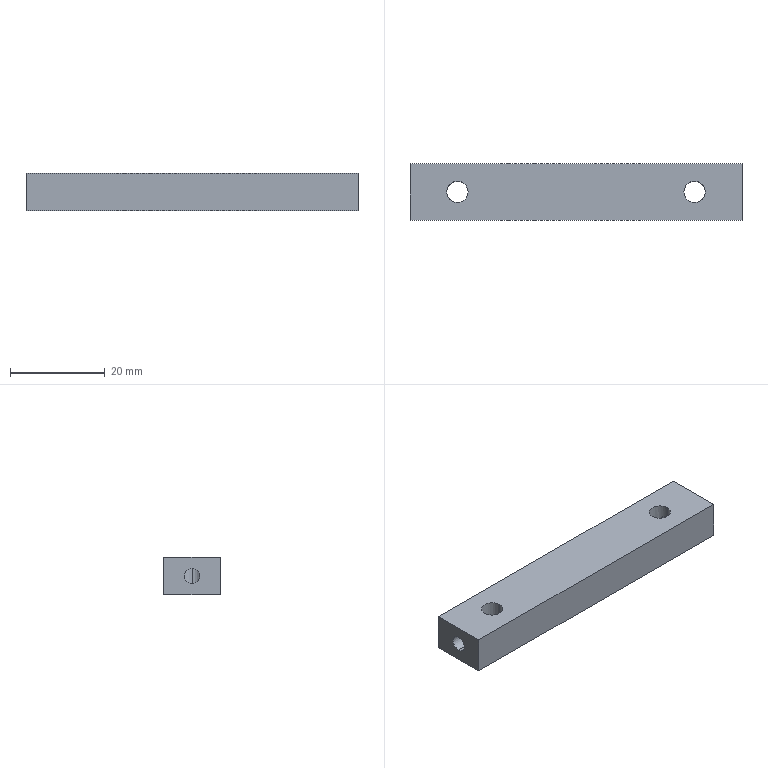Component | SolidWorks | InnerBagLiftingAluminumBlockB-1 | 1 solid | 14 faces | box 70 x 12 x 8 mm | volume 6330 mm3 | cylinder 8 | plane 6 | commonest cylinder face diameters 3.3 x4 4.5 x4
build123d program:
from build123d import *

# Parameters (mm, degrees)
SKETCH1_W             = 70
SKETCH1_H             = 12
BOSS_EXTRUDE1_DEPTH   = 4
SKETCH2_R             = 2.25
CUT_EXTRUDE1_DEPTH    = 8
M4_TAPPED_HOLE1_D     = 3.3
M4_TAPPED_HOLE1_DEPTH = 10.1
M4_TAPPED_HOLE1_TIP   = 1.65
M4_TAPPED_HOLE2_D     = 3.3
M4_TAPPED_HOLE2_DEPTH = 10.1
M4_TAPPED_HOLE2_TIP   = 1.65


with BuildPart() as part:
    # Sketch1 → Boss-Extrude1 (new, symmetric)
    with BuildSketch(Plane.XY):
        with Locations((35, 6)):
            Rectangle(SKETCH1_W, SKETCH1_H)
    extrude(amount=BOSS_EXTRUDE1_DEPTH, both=True)

    # Sketch2 → Cut-Extrude1 (cut)
    with BuildSketch(Plane.XY.offset(4)):
        with Locations((10, 6)):
            Circle(SKETCH2_R)
        with Locations((60, 6)):
            Circle(SKETCH2_R)
    extrude(amount=-CUT_EXTRUDE1_DEPTH, mode=Mode.SUBTRACT)

    # M4 Tapped Hole1
    with Locations(Plane(origin=(70, 6, 0), x_dir=(0, 0, 1), z_dir=(1, 0, 0))):
        with Locations((0, 0)):
            Hole(M4_TAPPED_HOLE1_D / 2, depth=M4_TAPPED_HOLE1_DEPTH)
            with Locations((0, 0, -(M4_TAPPED_HOLE1_DEPTH + M4_TAPPED_HOLE1_TIP / 2))):  # 90° drill point
                Cone(0, M4_TAPPED_HOLE1_D / 2, M4_TAPPED_HOLE1_TIP, mode=Mode.SUBTRACT)

    # M4 Tapped Hole2
    with Locations(Plane(origin=(0, 6, 0), x_dir=(0, 0, -1), z_dir=(-1, 0, 0))):
        with Locations((0, 0)):
            Hole(M4_TAPPED_HOLE2_D / 2, depth=M4_TAPPED_HOLE2_DEPTH)
            with Locations((0, 0, -(M4_TAPPED_HOLE2_DEPTH + M4_TAPPED_HOLE2_TIP / 2))):  # 90° drill point
                Cone(0, M4_TAPPED_HOLE2_D / 2, M4_TAPPED_HOLE2_TIP, mode=Mode.SUBTRACT)


solid = part.part

# Placed as in the assembly
solid = solid.moved(Location((29.354, -54.068, 191.933), (0, 0, 0)))
STEP:
#1=CARTESIAN_POINT('',(1.461,-1.892,7.491));
#2=VERTEX_POINT('',#1);
#3=CARTESIAN_POINT('',(1.461,-1.892,7.621));
#4=VERTEX_POINT('',#3);
#5=CARTESIAN_POINT('',(1.461,-1.892,7.491));
#6=CARTESIAN_POINT('',(1.461,-1.897,7.491));
#7=CARTESIAN_POINT('',(1.461,-1.901,7.492));
#8=CARTESIAN_POINT('',(1.462,-1.91,7.494));
#9=CARTESIAN_POINT('',(1.463,-1.914,7.495));
#10=CARTESIAN_POINT('',(1.467,-1.926,7.5));
#11=CARTESIAN_POINT('',(1.47,-1.933,7.505));
#12=CARTESIAN_POINT('',(1.477,-1.944,7.517));
#13=CARTESIAN_POINT('',(1.481,-1.949,7.523));
#14=CARTESIAN_POINT('',(1.487,-1.955,7.539));
#15=CARTESIAN_POINT('',(1.489,-1.957,7.547));
#16=CARTESIAN_POINT('',(1.489,-1.957,7.565));
#17=CARTESIAN_POINT('',(1.487,-1.955,7.574));
#18=CARTESIAN_POINT('',(1.483,-1.951,7.586));
#19=CARTESIAN_POINT('',(1.481,-1.949,7.589));
#20=CARTESIAN_POINT('',(1.477,-1.944,7.596));
#21=CARTESIAN_POINT('',(1.476,-1.941,7.599));
#22=CARTESIAN_POINT('',(1.472,-1.936,7.605));
#23=CARTESIAN_POINT('',(1.47,-1.933,7.608));
#24=CARTESIAN_POINT('',(1.467,-1.926,7.612));
#25=CARTESIAN_POINT('',(1.466,-1.922,7.614));
#26=CARTESIAN_POINT('',(1.462,-1.91,7.619));
#27=CARTESIAN_POINT('',(1.461,-1.901,7.621));
#28=CARTESIAN_POINT('',(1.461,-1.892,7.621));
#29=B_SPLINE_CURVE_WITH_KNOTS('',3,(#5,#6,#7,#8,#9,#10,#11,#12,#13,#14,#15,#16,#17,#18,#19,#20,#21,#22,#23,#24,#25,#26,#27,#28),.UNSPECIFIED.,.F.,.F.,(4,2,2,2,2,2,2,2,2,2,2,4),(0.005391,0.005727,0.006063,0.006736,0.007408,0.008081,0.008754,0.00909,0.009426,0.009762,0.0101,0.01077),.UNSPECIFIED.);
#30=EDGE_CURVE('',#2,#4,#29,.T.);
#31=ORIENTED_EDGE('',*,*,#30,.F.);
#32=CARTESIAN_POINT('',(1.156,-1.892,7.491));
#33=VERTEX_POINT('',#32);
#34=CARTESIAN_POINT('',(1.156,-1.892,7.491));
#35=DIRECTION('',(-1.,0.,0.));
#36=VECTOR('',#35,39.37);
#37=LINE('',#34,#36);
#38=EDGE_CURVE('',#2,#33,#37,.T.);
#39=ORIENTED_EDGE('',*,*,#38,.T.);
#40=CARTESIAN_POINT('',(1.156,-1.892,7.621));
#41=VERTEX_POINT('',#40);
#42=CARTESIAN_POINT('',(1.156,-1.892,7.556));
#43=DIRECTION('',(-1.,0.,0.));
#44=DIRECTION('',(0.,0.,1.));
#45=AXIS2_PLACEMENT_3D('',#42,#43,#44);
#46=CIRCLE('',#45,0.06496);
#47=EDGE_CURVE('',#33,#41,#46,.T.);
#48=ORIENTED_EDGE('',*,*,#47,.T.);
#49=CARTESIAN_POINT('',(1.156,-1.892,7.621));
#50=DIRECTION('',(-1.,0.,0.));
#51=VECTOR('',#50,39.37);
#52=LINE('',#49,#51);
#53=EDGE_CURVE('',#4,#41,#52,.T.);
#54=ORIENTED_EDGE('',*,*,#53,.F.);
#55=EDGE_LOOP('',(#31,#39,#48,#54));
#56=FACE_OUTER_BOUND('',#55,.T.);
#57=CARTESIAN_POINT('',(1.156,-1.892,7.556));
#58=DIRECTION('',(-1.,0.,0.));
#59=DIRECTION('',(0.,0.,1.));
#60=AXIS2_PLACEMENT_3D('',#57,#58,#59);
#61=CYLINDRICAL_SURFACE('',#60,0.06496);
#62=ADVANCED_FACE('',(#56),#61,.F.);
#63=CARTESIAN_POINT('',(3.606,-1.892,7.621));
#64=VERTEX_POINT('',#63);
#65=CARTESIAN_POINT('',(3.606,-1.892,7.491));
#66=VERTEX_POINT('',#65);
#67=CARTESIAN_POINT('',(3.606,-1.892,7.621));
#68=CARTESIAN_POINT('',(3.606,-1.897,7.621));
#69=CARTESIAN_POINT('',(3.606,-1.901,7.621));
#70=CARTESIAN_POINT('',(3.605,-1.91,7.619));
#71=CARTESIAN_POINT('',(3.604,-1.914,7.618));
#72=CARTESIAN_POINT('',(3.6,-1.926,7.613));
#73=CARTESIAN_POINT('',(3.597,-1.933,7.608));
#74=CARTESIAN_POINT('',(3.59,-1.944,7.596));
#75=CARTESIAN_POINT('',(3.586,-1.949,7.589));
#76=CARTESIAN_POINT('',(3.58,-1.955,7.574));
#77=CARTESIAN_POINT('',(3.578,-1.957,7.565));
#78=CARTESIAN_POINT('',(3.578,-1.957,7.547));
#79=CARTESIAN_POINT('',(3.58,-1.955,7.539));
#80=CARTESIAN_POINT('',(3.585,-1.951,7.527));
#81=CARTESIAN_POINT('',(3.586,-1.949,7.524));
#82=CARTESIAN_POINT('',(3.59,-1.944,7.517));
#83=CARTESIAN_POINT('',(3.592,-1.941,7.514));
#84=CARTESIAN_POINT('',(3.595,-1.936,7.508));
#85=CARTESIAN_POINT('',(3.597,-1.933,7.505));
#86=CARTESIAN_POINT('',(3.6,-1.926,7.5));
#87=CARTESIAN_POINT('',(3.601,-1.922,7.498));
#88=CARTESIAN_POINT('',(3.605,-1.91,7.493));
#89=CARTESIAN_POINT('',(3.606,-1.901,7.491));
#90=CARTESIAN_POINT('',(3.606,-1.892,7.491));
#91=B_SPLINE_CURVE_WITH_KNOTS('',3,(#67,#68,#69,#70,#71,#72,#73,#74,#75,#76,#77,#78,#79,#80,#81,#82,#83,#84,#85,#86,#87,#88,#89,#90),.UNSPECIFIED.,.F.,.F.,(4,2,2,2,2,2,2,2,2,2,2,4),(0.005391,0.005727,0.006063,0.006736,0.007408,0.008081,0.008754,0.00909,0.009426,0.009762,0.0101,0.01077),.UNSPECIFIED.);
#92=EDGE_CURVE('',#64,#66,#91,.T.);
#93=ORIENTED_EDGE('',*,*,#92,.F.);
#94=CARTESIAN_POINT('',(3.912,-1.892,7.621));
#95=VERTEX_POINT('',#94);
#96=CARTESIAN_POINT('',(3.912,-1.892,7.621));
#97=DIRECTION('',(1.,0.,0.));
#98=VECTOR('',#97,39.37);
#99=LINE('',#96,#98);
#100=EDGE_CURVE('',#64,#95,#99,.T.);
#101=ORIENTED_EDGE('',*,*,#100,.T.);
#102=CARTESIAN_POINT('',(3.912,-1.892,7.491));
#103=VERTEX_POINT('',#102);
#104=CARTESIAN_POINT('',(3.912,-1.892,7.556));
#105=DIRECTION('',(1.,0.,0.));
#106=DIRECTION('',(0.,0.,-1.));
#107=AXIS2_PLACEMENT_3D('',#104,#105,#106);
#108=CIRCLE('',#107,0.06496);
#109=EDGE_CURVE('',#95,#103,#108,.T.);
#110=ORIENTED_EDGE('',*,*,#109,.T.);
#111=CARTESIAN_POINT('',(3.912,-1.892,7.491));
#112=DIRECTION('',(1.,0.,0.));
#113=VECTOR('',#112,39.37);
#114=LINE('',#111,#113);
#115=EDGE_CURVE('',#66,#103,#114,.T.);
#116=ORIENTED_EDGE('',*,*,#115,.F.);
#117=EDGE_LOOP('',(#93,#101,#110,#116));
#118=FACE_OUTER_BOUND('',#117,.T.);
#119=CARTESIAN_POINT('',(3.912,-1.892,7.556));
#120=DIRECTION('',(1.,0.,0.));
#121=DIRECTION('',(0.,0.,-1.));
#122=AXIS2_PLACEMENT_3D('',#119,#120,#121);
#123=CYLINDRICAL_SURFACE('',#122,0.06496);
#124=ADVANCED_FACE('',(#118),#123,.F.);
#125=CARTESIAN_POINT('',(3.429,-1.892,7.399));
#126=VERTEX_POINT('',#125);
#127=CARTESIAN_POINT('',(3.606,-1.892,7.399));
#128=VERTEX_POINT('',#127);
#129=CARTESIAN_POINT('',(3.518,-1.892,7.399));
#130=DIRECTION('',(0.,0.,1.));
#131=DIRECTION('',(1.,0.,0.));
#132=AXIS2_PLACEMENT_3D('',#129,#130,#131);
#133=CIRCLE('',#132,0.08858);
#134=EDGE_CURVE('',#126,#128,#133,.T.);
#135=ORIENTED_EDGE('',*,*,#134,.F.);
#136=CARTESIAN_POINT('',(3.429,-1.892,7.714));
#137=VERTEX_POINT('',#136);
#138=CARTESIAN_POINT('',(3.429,-1.892,7.399));
#139=DIRECTION('',(0.,0.,1.));
#140=VECTOR('',#139,39.37);
#141=LINE('',#138,#140);
#142=EDGE_CURVE('',#126,#137,#141,.T.);
#143=ORIENTED_EDGE('',*,*,#142,.T.);
#144=CARTESIAN_POINT('',(3.606,-1.892,7.714));
#145=VERTEX_POINT('',#144);
#146=CARTESIAN_POINT('',(3.518,-1.892,7.714));
#147=DIRECTION('',(0.,0.,1.));
#148=DIRECTION('',(1.,0.,0.));
#149=AXIS2_PLACEMENT_3D('',#146,#147,#148);
#150=CIRCLE('',#149,0.08858);
#151=EDGE_CURVE('',#137,#145,#150,.T.);
#152=ORIENTED_EDGE('',*,*,#151,.T.);
#153=CARTESIAN_POINT('',(3.606,-1.892,7.399));
#154=DIRECTION('',(0.,0.,1.));
#155=VECTOR('',#154,39.37);
#156=LINE('',#153,#155);
#157=EDGE_CURVE('',#64,#145,#156,.T.);
#158=ORIENTED_EDGE('',*,*,#157,.F.);
#159=ORIENTED_EDGE('',*,*,#92,.T.);
#160=CARTESIAN_POINT('',(3.606,-1.892,7.399));
#161=DIRECTION('',(0.,0.,1.));
#162=VECTOR('',#161,39.37);
#163=LINE('',#160,#162);
#164=EDGE_CURVE('',#128,#66,#163,.T.);
#165=ORIENTED_EDGE('',*,*,#164,.F.);
#166=EDGE_LOOP('',(#135,#143,#152,#158,#159,#165));
#167=FACE_OUTER_BOUND('',#166,.T.);
#168=CARTESIAN_POINT('',(3.518,-1.892,7.399));
#169=DIRECTION('',(0.,0.,1.));
#170=DIRECTION('',(1.,0.,0.));
#171=AXIS2_PLACEMENT_3D('',#168,#169,#170);
#172=CYLINDRICAL_SURFACE('',#171,0.08858);
#173=ADVANCED_FACE('',(#167),#172,.F.);
#174=CARTESIAN_POINT('',(1.461,-1.892,7.399));
#175=VERTEX_POINT('',#174);
#176=CARTESIAN_POINT('',(1.638,-1.892,7.399));
#177=VERTEX_POINT('',#176);
#178=CARTESIAN_POINT('',(1.549,-1.892,7.399));
#179=DIRECTION('',(0.,0.,1.));
#180=DIRECTION('',(1.,0.,0.));
#181=AXIS2_PLACEMENT_3D('',#178,#179,#180);
#182=CIRCLE('',#181,0.08858);
#183=EDGE_CURVE('',#175,#177,#182,.T.);
#184=ORIENTED_EDGE('',*,*,#183,.F.);
#185=CARTESIAN_POINT('',(1.461,-1.892,7.399));
#186=DIRECTION('',(0.,0.,1.));
#187=VECTOR('',#186,39.37);
#188=LINE('',#185,#187);
#189=EDGE_CURVE('',#175,#2,#188,.T.);
#190=ORIENTED_EDGE('',*,*,#189,.T.);
#191=ORIENTED_EDGE('',*,*,#30,.T.);
#192=CARTESIAN_POINT('',(1.461,-1.892,7.714));
#193=VERTEX_POINT('',#192);
#194=CARTESIAN_POINT('',(1.461,-1.892,7.399));
#195=DIRECTION('',(0.,0.,1.));
#196=VECTOR('',#195,39.37);
#197=LINE('',#194,#196);
#198=EDGE_CURVE('',#4,#193,#197,.T.);
#199=ORIENTED_EDGE('',*,*,#198,.T.);
#200=CARTESIAN_POINT('',(1.638,-1.892,7.714));
#201=VERTEX_POINT('',#200);
#202=CARTESIAN_POINT('',(1.549,-1.892,7.714));
#203=DIRECTION('',(0.,0.,1.));
#204=DIRECTION('',(1.,0.,0.));
#205=AXIS2_PLACEMENT_3D('',#202,#203,#204);
#206=CIRCLE('',#205,0.08858);
#207=EDGE_CURVE('',#193,#201,#206,.T.);
#208=ORIENTED_EDGE('',*,*,#207,.T.);
#209=CARTESIAN_POINT('',(1.638,-1.892,7.399));
#210=DIRECTION('',(0.,0.,1.));
#211=VECTOR('',#210,39.37);
#212=LINE('',#209,#211);
#213=EDGE_CURVE('',#177,#201,#212,.T.);
#214=ORIENTED_EDGE('',*,*,#213,.F.);
#215=EDGE_LOOP('',(#184,#190,#191,#199,#208,#214));
#216=FACE_OUTER_BOUND('',#215,.T.);
#217=CARTESIAN_POINT('',(1.549,-1.892,7.399));
#218=DIRECTION('',(0.,0.,1.));
#219=DIRECTION('',(1.,0.,0.));
#220=AXIS2_PLACEMENT_3D('',#217,#218,#219);
#221=CYLINDRICAL_SURFACE('',#220,0.08858);
#222=ADVANCED_FACE('',(#216),#221,.F.);
#223=CARTESIAN_POINT('',(1.156,-1.892,7.556));
#224=DIRECTION('',(-1.,0.,0.));
#225=DIRECTION('',(0.,0.,1.));
#226=AXIS2_PLACEMENT_3D('',#223,#224,#225);
#227=CIRCLE('',#226,0.06496);
#228=EDGE_CURVE('',#41,#33,#227,.T.);
#229=ORIENTED_EDGE('',*,*,#228,.F.);
#230=ORIENTED_EDGE('',*,*,#47,.F.);
#231=EDGE_LOOP('',(#229,#230));
#232=FACE_BOUND('',#231,.T.);
#233=CARTESIAN_POINT('',(1.156,-1.656,7.399));
#234=VERTEX_POINT('',#233);
#235=CARTESIAN_POINT('',(1.156,-2.129,7.399));
#236=VERTEX_POINT('',#235);
#237=CARTESIAN_POINT('',(1.156,-2.129,7.399));
#238=DIRECTION('',(0.,-1.,0.));
#239=VECTOR('',#238,39.37);
#240=LINE('',#237,#239);
#241=EDGE_CURVE('',#234,#236,#240,.T.);
#242=ORIENTED_EDGE('',*,*,#241,.T.);
#243=CARTESIAN_POINT('',(1.156,-2.129,7.714));
#244=VERTEX_POINT('',#243);
#245=CARTESIAN_POINT('',(1.156,-2.129,7.714));
#246=DIRECTION('',(0.,0.,-1.));
#247=VECTOR('',#246,39.37);
#248=LINE('',#245,#247);
#249=EDGE_CURVE('',#244,#236,#248,.T.);
#250=ORIENTED_EDGE('',*,*,#249,.F.);
#251=CARTESIAN_POINT('',(1.156,-1.656,7.714));
#252=VERTEX_POINT('',#251);
#253=CARTESIAN_POINT('',(1.156,-2.129,7.714));
#254=DIRECTION('',(0.,-1.,0.));
#255=VECTOR('',#254,39.37);
#256=LINE('',#253,#255);
#257=EDGE_CURVE('',#252,#244,#256,.T.);
#258=ORIENTED_EDGE('',*,*,#257,.F.);
#259=CARTESIAN_POINT('',(1.156,-1.656,7.714));
#260=DIRECTION('',(0.,0.,-1.));
#261=VECTOR('',#260,39.37);
#262=LINE('',#259,#261);
#263=EDGE_CURVE('',#252,#234,#262,.T.);
#264=ORIENTED_EDGE('',*,*,#263,.T.);
#265=EDGE_LOOP('',(#242,#250,#258,#264));
#266=FACE_OUTER_BOUND('',#265,.T.);
#267=CARTESIAN_POINT('',(1.156,-2.129,7.714));
#268=DIRECTION('',(1.,0.,0.));
#269=DIRECTION('',(0.,0.,-1.));
#270=AXIS2_PLACEMENT_3D('',#267,#268,#269);
#271=PLANE('',#270);
#272=ADVANCED_FACE('',(#232,#266),#271,.F.);
#273=CARTESIAN_POINT('',(3.912,-2.129,7.399));
#274=VERTEX_POINT('',#273);
#275=CARTESIAN_POINT('',(1.156,-2.129,7.399));
#276=DIRECTION('',(1.,0.,0.));
#277=VECTOR('',#276,39.37);
#278=LINE('',#275,#277);
#279=EDGE_CURVE('',#236,#274,#278,.T.);
#280=ORIENTED_EDGE('',*,*,#279,.T.);
#281=CARTESIAN_POINT('',(3.912,-2.129,7.714));
#282=VERTEX_POINT('',#281);
#283=CARTESIAN_POINT('',(3.912,-2.129,7.714));
#284=DIRECTION('',(0.,0.,-1.));
#285=VECTOR('',#284,39.37);
#286=LINE('',#283,#285);
#287=EDGE_CURVE('',#282,#274,#286,.T.);
#288=ORIENTED_EDGE('',*,*,#287,.F.);
#289=CARTESIAN_POINT('',(1.156,-2.129,7.714));
#290=DIRECTION('',(1.,0.,0.));
#291=VECTOR('',#290,39.37);
#292=LINE('',#289,#291);
#293=EDGE_CURVE('',#244,#282,#292,.T.);
#294=ORIENTED_EDGE('',*,*,#293,.F.);
#295=ORIENTED_EDGE('',*,*,#249,.T.);
#296=EDGE_LOOP('',(#280,#288,#294,#295));
#297=FACE_OUTER_BOUND('',#296,.T.);
#298=CARTESIAN_POINT('',(1.156,-2.129,7.714));
#299=DIRECTION('',(0.,1.,0.));
#300=DIRECTION('',(0.,0.,1.));
#301=AXIS2_PLACEMENT_3D('',#298,#299,#300);
#302=PLANE('',#301);
#303=ADVANCED_FACE('',(#297),#302,.F.);
#304=CARTESIAN_POINT('',(3.912,-1.892,7.556));
#305=DIRECTION('',(1.,0.,0.));
#306=DIRECTION('',(0.,0.,-1.));
#307=AXIS2_PLACEMENT_3D('',#304,#305,#306);
#308=CIRCLE('',#307,0.06496);
#309=EDGE_CURVE('',#103,#95,#308,.T.);
#310=ORIENTED_EDGE('',*,*,#309,.F.);
#311=ORIENTED_EDGE('',*,*,#109,.F.);
#312=EDGE_LOOP('',(#310,#311));
#313=FACE_BOUND('',#312,.T.);
#314=CARTESIAN_POINT('',(3.912,-1.656,7.399));
#315=VERTEX_POINT('',#314);
#316=CARTESIAN_POINT('',(3.912,-2.129,7.399));
#317=DIRECTION('',(0.,1.,0.));
#318=VECTOR('',#317,39.37);
#319=LINE('',#316,#318);
#320=EDGE_CURVE('',#274,#315,#319,.T.);
#321=ORIENTED_EDGE('',*,*,#320,.T.);
#322=CARTESIAN_POINT('',(3.912,-1.656,7.714));
#323=VERTEX_POINT('',#322);
#324=CARTESIAN_POINT('',(3.912,-1.656,7.714));
#325=DIRECTION('',(0.,0.,-1.));
#326=VECTOR('',#325,39.37);
#327=LINE('',#324,#326);
#328=EDGE_CURVE('',#323,#315,#327,.T.);
#329=ORIENTED_EDGE('',*,*,#328,.F.);
#330=CARTESIAN_POINT('',(3.912,-2.129,7.714));
#331=DIRECTION('',(0.,1.,0.));
#332=VECTOR('',#331,39.37);
#333=LINE('',#330,#332);
#334=EDGE_CURVE('',#282,#323,#333,.T.);
#335=ORIENTED_EDGE('',*,*,#334,.F.);
#336=ORIENTED_EDGE('',*,*,#287,.T.);
#337=EDGE_LOOP('',(#321,#329,#335,#336));
#338=FACE_OUTER_BOUND('',#337,.T.);
#339=CARTESIAN_POINT('',(3.912,-2.129,7.714));
#340=DIRECTION('',(-1.,0.,0.));
#341=DIRECTION('',(0.,0.,1.));
#342=AXIS2_PLACEMENT_3D('',#339,#340,#341);
#343=PLANE('',#342);
#344=ADVANCED_FACE('',(#313,#338),#343,.F.);
#345=CARTESIAN_POINT('',(1.156,-1.656,7.399));
#346=DIRECTION('',(-1.,0.,0.));
#347=VECTOR('',#346,39.37);
#348=LINE('',#345,#347);
#349=EDGE_CURVE('',#315,#234,#348,.T.);
#350=ORIENTED_EDGE('',*,*,#349,.T.);
#351=ORIENTED_EDGE('',*,*,#263,.F.);
#352=CARTESIAN_POINT('',(1.156,-1.656,7.714));
#353=DIRECTION('',(-1.,0.,0.));
#354=VECTOR('',#353,39.37);
#355=LINE('',#352,#354);
#356=EDGE_CURVE('',#323,#252,#355,.T.);
#357=ORIENTED_EDGE('',*,*,#356,.F.);
#358=ORIENTED_EDGE('',*,*,#328,.T.);
#359=EDGE_LOOP('',(#350,#351,#357,#358));
#360=FACE_OUTER_BOUND('',#359,.T.);
#361=CARTESIAN_POINT('',(1.156,-1.656,7.714));
#362=DIRECTION('',(0.,-1.,0.));
#363=DIRECTION('',(0.,0.,-1.));
#364=AXIS2_PLACEMENT_3D('',#361,#362,#363);
#365=PLANE('',#364);
#366=ADVANCED_FACE('',(#360),#365,.F.);
#367=CARTESIAN_POINT('',(3.518,-1.892,7.714));
#368=DIRECTION('',(0.,0.,1.));
#369=DIRECTION('',(1.,0.,0.));
#370=AXIS2_PLACEMENT_3D('',#367,#368,#369);
#371=CIRCLE('',#370,0.08858);
#372=EDGE_CURVE('',#145,#137,#371,.T.);
#373=ORIENTED_EDGE('',*,*,#372,.F.);
#374=ORIENTED_EDGE('',*,*,#151,.F.);
#375=EDGE_LOOP('',(#373,#374));
#376=FACE_BOUND('',#375,.T.);
#377=CARTESIAN_POINT('',(1.549,-1.892,7.714));
#378=DIRECTION('',(0.,0.,1.));
#379=DIRECTION('',(1.,0.,0.));
#380=AXIS2_PLACEMENT_3D('',#377,#378,#379);
#381=CIRCLE('',#380,0.08858);
#382=EDGE_CURVE('',#201,#193,#381,.T.);
#383=ORIENTED_EDGE('',*,*,#382,.F.);
#384=ORIENTED_EDGE('',*,*,#207,.F.);
#385=EDGE_LOOP('',(#383,#384));
#386=FACE_BOUND('',#385,.T.);
#387=ORIENTED_EDGE('',*,*,#257,.T.);
#388=ORIENTED_EDGE('',*,*,#293,.T.);
#389=ORIENTED_EDGE('',*,*,#334,.T.);
#390=ORIENTED_EDGE('',*,*,#356,.T.);
#391=EDGE_LOOP('',(#387,#388,#389,#390));
#392=FACE_OUTER_BOUND('',#391,.T.);
#393=CARTESIAN_POINT('',(1.156,-2.129,7.714));
#394=DIRECTION('',(0.,0.,-1.));
#395=DIRECTION('',(-1.,0.,0.));
#396=AXIS2_PLACEMENT_3D('',#393,#394,#395);
#397=PLANE('',#396);
#398=ADVANCED_FACE('',(#376,#386,#392),#397,.F.);
#399=CARTESIAN_POINT('',(3.518,-1.892,7.399));
#400=DIRECTION('',(0.,0.,1.));
#401=DIRECTION('',(1.,0.,0.));
#402=AXIS2_PLACEMENT_3D('',#399,#400,#401);
#403=CIRCLE('',#402,0.08858);
#404=EDGE_CURVE('',#128,#126,#403,.T.);
#405=ORIENTED_EDGE('',*,*,#404,.T.);
#406=ORIENTED_EDGE('',*,*,#134,.T.);
#407=EDGE_LOOP('',(#405,#406));
#408=FACE_BOUND('',#407,.T.);
#409=CARTESIAN_POINT('',(1.549,-1.892,7.399));
#410=DIRECTION('',(0.,0.,1.));
#411=DIRECTION('',(1.,0.,0.));
#412=AXIS2_PLACEMENT_3D('',#409,#410,#411);
#413=CIRCLE('',#412,0.08858);
#414=EDGE_CURVE('',#177,#175,#413,.T.);
#415=ORIENTED_EDGE('',*,*,#414,.T.);
#416=ORIENTED_EDGE('',*,*,#183,.T.);
#417=EDGE_LOOP('',(#415,#416));
#418=FACE_BOUND('',#417,.T.);
#419=ORIENTED_EDGE('',*,*,#241,.F.);
#420=ORIENTED_EDGE('',*,*,#349,.F.);
#421=ORIENTED_EDGE('',*,*,#320,.F.);
#422=ORIENTED_EDGE('',*,*,#279,.F.);
#423=EDGE_LOOP('',(#419,#420,#421,#422));
#424=FACE_OUTER_BOUND('',#423,.T.);
#425=CARTESIAN_POINT('',(1.156,-2.129,7.399));
#426=DIRECTION('',(0.,0.,-1.));
#427=DIRECTION('',(-1.,0.,0.));
#428=AXIS2_PLACEMENT_3D('',#425,#426,#427);
#429=PLANE('',#428);
#430=ADVANCED_FACE('',(#408,#418,#424),#429,.T.);
#431=ORIENTED_EDGE('',*,*,#189,.F.);
#432=ORIENTED_EDGE('',*,*,#414,.F.);
#433=ORIENTED_EDGE('',*,*,#213,.T.);
#434=ORIENTED_EDGE('',*,*,#382,.T.);
#435=ORIENTED_EDGE('',*,*,#198,.F.);
#436=CARTESIAN_POINT('',(1.461,-1.892,7.621));
#437=CARTESIAN_POINT('',(1.461,-1.888,7.621));
#438=CARTESIAN_POINT('',(1.461,-1.884,7.621));
#439=CARTESIAN_POINT('',(1.462,-1.875,7.619));
#440=CARTESIAN_POINT('',(1.463,-1.871,7.618));
#441=CARTESIAN_POINT('',(1.467,-1.859,7.613));
#442=CARTESIAN_POINT('',(1.47,-1.852,7.608));
#443=CARTESIAN_POINT('',(1.476,-1.843,7.599));
#444=CARTESIAN_POINT('',(1.477,-1.841,7.596));
#445=CARTESIAN_POINT('',(1.481,-1.836,7.589));
#446=CARTESIAN_POINT('',(1.483,-1.834,7.586));
#447=CARTESIAN_POINT('',(1.486,-1.831,7.578));
#448=CARTESIAN_POINT('',(1.487,-1.83,7.574));
#449=CARTESIAN_POINT('',(1.489,-1.828,7.565));
#450=CARTESIAN_POINT('',(1.489,-1.827,7.561));
#451=CARTESIAN_POINT('',(1.489,-1.827,7.552));
#452=CARTESIAN_POINT('',(1.489,-1.828,7.547));
#453=CARTESIAN_POINT('',(1.487,-1.83,7.539));
#454=CARTESIAN_POINT('',(1.486,-1.831,7.535));
#455=CARTESIAN_POINT('',(1.481,-1.836,7.523));
#456=CARTESIAN_POINT('',(1.477,-1.84,7.517));
#457=CARTESIAN_POINT('',(1.47,-1.852,7.505));
#458=CARTESIAN_POINT('',(1.467,-1.859,7.5));
#459=CARTESIAN_POINT('',(1.463,-1.871,7.495));
#460=CARTESIAN_POINT('',(1.462,-1.875,7.494));
#461=CARTESIAN_POINT('',(1.461,-1.883,7.492));
#462=CARTESIAN_POINT('',(1.461,-1.888,7.491));
#463=CARTESIAN_POINT('',(1.461,-1.892,7.491));
#464=B_SPLINE_CURVE_WITH_KNOTS('',3,(#436,#437,#438,#439,#440,#441,#442,#443,#444,#445,#446,#447,#448,#449,#450,#451,#452,#453,#454,#455,#456,#457,#458,#459,#460,#461,#462,#463),.UNSPECIFIED.,.F.,.F.,(4,2,2,2,2,2,2,2,2,2,2,2,2,4),(0.,0.0003369,0.0006738,0.001348,0.001685,0.002022,0.002358,0.002695,0.003032,0.003369,0.004043,0.004717,0.005054,0.005391),.UNSPECIFIED.);
#465=EDGE_CURVE('',#4,#2,#464,.T.);
#466=ORIENTED_EDGE('',*,*,#465,.T.);
#467=EDGE_LOOP('',(#431,#432,#433,#434,#435,#466));
#468=FACE_OUTER_BOUND('',#467,.T.);
#469=CARTESIAN_POINT('',(1.549,-1.892,7.399));
#470=DIRECTION('',(0.,0.,1.));
#471=DIRECTION('',(1.,0.,0.));
#472=AXIS2_PLACEMENT_3D('',#469,#470,#471);
#473=CYLINDRICAL_SURFACE('',#472,0.08858);
#474=ADVANCED_FACE('',(#468),#473,.F.);
#475=ORIENTED_EDGE('',*,*,#142,.F.);
#476=ORIENTED_EDGE('',*,*,#404,.F.);
#477=ORIENTED_EDGE('',*,*,#164,.T.);
#478=CARTESIAN_POINT('',(3.606,-1.892,7.491));
#479=CARTESIAN_POINT('',(3.606,-1.888,7.491));
#480=CARTESIAN_POINT('',(3.606,-1.884,7.492));
#481=CARTESIAN_POINT('',(3.605,-1.875,7.494));
#482=CARTESIAN_POINT('',(3.604,-1.871,7.495));
#483=CARTESIAN_POINT('',(3.6,-1.859,7.5));
#484=CARTESIAN_POINT('',(3.597,-1.852,7.505));
#485=CARTESIAN_POINT('',(3.592,-1.843,7.514));
#486=CARTESIAN_POINT('',(3.59,-1.841,7.517));
#487=CARTESIAN_POINT('',(3.586,-1.836,7.524));
#488=CARTESIAN_POINT('',(3.585,-1.834,7.527));
#489=CARTESIAN_POINT('',(3.582,-1.831,7.535));
#490=CARTESIAN_POINT('',(3.58,-1.83,7.539));
#491=CARTESIAN_POINT('',(3.579,-1.828,7.548));
#492=CARTESIAN_POINT('',(3.578,-1.827,7.552));
#493=CARTESIAN_POINT('',(3.578,-1.827,7.561));
#494=CARTESIAN_POINT('',(3.579,-1.828,7.565));
#495=CARTESIAN_POINT('',(3.58,-1.83,7.574));
#496=CARTESIAN_POINT('',(3.582,-1.831,7.578));
#497=CARTESIAN_POINT('',(3.586,-1.836,7.59));
#498=CARTESIAN_POINT('',(3.59,-1.84,7.596));
#499=CARTESIAN_POINT('',(3.597,-1.852,7.608));
#500=CARTESIAN_POINT('',(3.6,-1.859,7.613));
#501=CARTESIAN_POINT('',(3.604,-1.871,7.618));
#502=CARTESIAN_POINT('',(3.605,-1.875,7.619));
#503=CARTESIAN_POINT('',(3.606,-1.883,7.621));
#504=CARTESIAN_POINT('',(3.606,-1.888,7.621));
#505=CARTESIAN_POINT('',(3.606,-1.892,7.621));
#506=B_SPLINE_CURVE_WITH_KNOTS('',3,(#478,#479,#480,#481,#482,#483,#484,#485,#486,#487,#488,#489,#490,#491,#492,#493,#494,#495,#496,#497,#498,#499,#500,#501,#502,#503,#504,#505),.UNSPECIFIED.,.F.,.F.,(4,2,2,2,2,2,2,2,2,2,2,2,2,4),(0.,0.0003369,0.0006738,0.001348,0.001685,0.002022,0.002358,0.002695,0.003032,0.003369,0.004043,0.004717,0.005054,0.005391),.UNSPECIFIED.);
#507=EDGE_CURVE('',#66,#64,#506,.T.);
#508=ORIENTED_EDGE('',*,*,#507,.T.);
#509=ORIENTED_EDGE('',*,*,#157,.T.);
#510=ORIENTED_EDGE('',*,*,#372,.T.);
#511=EDGE_LOOP('',(#475,#476,#477,#508,#509,#510));
#512=FACE_OUTER_BOUND('',#511,.T.);
#513=CARTESIAN_POINT('',(3.518,-1.892,7.399));
#514=DIRECTION('',(0.,0.,1.));
#515=DIRECTION('',(1.,0.,0.));
#516=AXIS2_PLACEMENT_3D('',#513,#514,#515);
#517=CYLINDRICAL_SURFACE('',#516,0.08858);
#518=ADVANCED_FACE('',(#512),#517,.F.);
#519=ORIENTED_EDGE('',*,*,#100,.F.);
#520=ORIENTED_EDGE('',*,*,#507,.F.);
#521=ORIENTED_EDGE('',*,*,#115,.T.);
#522=ORIENTED_EDGE('',*,*,#309,.T.);
#523=EDGE_LOOP('',(#519,#520,#521,#522));
#524=FACE_OUTER_BOUND('',#523,.T.);
#525=CARTESIAN_POINT('',(3.912,-1.892,7.556));
#526=DIRECTION('',(1.,0.,0.));
#527=DIRECTION('',(0.,0.,-1.));
#528=AXIS2_PLACEMENT_3D('',#525,#526,#527);
#529=CYLINDRICAL_SURFACE('',#528,0.06496);
#530=ADVANCED_FACE('',(#524),#529,.F.);
#531=ORIENTED_EDGE('',*,*,#38,.F.);
#532=ORIENTED_EDGE('',*,*,#465,.F.);
#533=ORIENTED_EDGE('',*,*,#53,.T.);
#534=ORIENTED_EDGE('',*,*,#228,.T.);
#535=EDGE_LOOP('',(#531,#532,#533,#534));
#536=FACE_OUTER_BOUND('',#535,.T.);
#537=CARTESIAN_POINT('',(1.156,-1.892,7.556));
#538=DIRECTION('',(-1.,0.,0.));
#539=DIRECTION('',(0.,0.,1.));
#540=AXIS2_PLACEMENT_3D('',#537,#538,#539);
#541=CYLINDRICAL_SURFACE('',#540,0.06496);
#542=ADVANCED_FACE('',(#536),#541,.F.);
#543=CLOSED_SHELL('',(#62,#124,#173,#222,#272,#303,#344,#366,#398,#430,#474,#518,#530,#542));
#544=MANIFOLD_SOLID_BREP('',#543);
#545=CARTESIAN_POINT('',(0.,0.,0.));
#546=DIRECTION('',(0.,0.,1.));
#547=DIRECTION('',(1.,0.,0.));
#548=AXIS2_PLACEMENT_3D('',#545,#546,#547);
#549=(LENGTH_UNIT()NAMED_UNIT(*)SI_UNIT($,.METRE.));
#550=LENGTH_MEASURE_WITH_UNIT(LENGTH_MEASURE(0.0254),#549);
#551=DIMENSIONAL_EXPONENTS(1.,0.,0.,0.,0.,0.,0.);
#552=(CONVERSION_BASED_UNIT('',#550)LENGTH_UNIT()NAMED_UNIT(#551));
#553=UNCERTAINTY_MEASURE_WITH_UNIT(LENGTH_MEASURE(0.00001),#552,'','');
#554=(NAMED_UNIT(*)PLANE_ANGLE_UNIT()SI_UNIT($,.RADIAN.));
#555=(NAMED_UNIT(*)SI_UNIT($,.STERADIAN.)SOLID_ANGLE_UNIT());
#556=(GEOMETRIC_REPRESENTATION_CONTEXT(3)GLOBAL_UNCERTAINTY_ASSIGNED_CONTEXT((#553))GLOBAL_UNIT_ASSIGNED_CONTEXT((#552,#554,#555))REPRESENTATION_CONTEXT('',''));
#557=ADVANCED_BREP_SHAPE_REPRESENTATION('',(#544,#548),#556);
#558=COLOUR_RGB('',0.7922,0.8196,0.9333);
#559=FILL_AREA_STYLE_COLOUR('',#558);
#560=FILL_AREA_STYLE('',(#559));
#561=SURFACE_STYLE_FILL_AREA(#560);
#562=SURFACE_SIDE_STYLE('',(#561));
#563=SURFACE_STYLE_USAGE(.BOTH.,#562);
#564=PRESENTATION_STYLE_ASSIGNMENT((#563));
#565=STYLED_ITEM('',(#564),#544);
#566=(LENGTH_UNIT()NAMED_UNIT(*)SI_UNIT($,.METRE.));
#567=LENGTH_MEASURE_WITH_UNIT(LENGTH_MEASURE(0.0254),#566);
#568=DIMENSIONAL_EXPONENTS(1.,0.,0.,0.,0.,0.,0.);
#569=(CONVERSION_BASED_UNIT('',#567)LENGTH_UNIT()NAMED_UNIT(#568));
#570=UNCERTAINTY_MEASURE_WITH_UNIT(LENGTH_MEASURE(0.00001),#569,'','');
#571=(NAMED_UNIT(*)PLANE_ANGLE_UNIT()SI_UNIT($,.RADIAN.));
#572=(NAMED_UNIT(*)SI_UNIT($,.STERADIAN.)SOLID_ANGLE_UNIT());
#573=(GEOMETRIC_REPRESENTATION_CONTEXT(3)GLOBAL_UNCERTAINTY_ASSIGNED_CONTEXT((#570))GLOBAL_UNIT_ASSIGNED_CONTEXT((#569,#571,#572))REPRESENTATION_CONTEXT('',''));
#574=MECHANICAL_DESIGN_GEOMETRIC_PRESENTATION_REPRESENTATION('',(#565),#573);
#575=PRESENTATION_LAYER_ASSIGNMENT('','',(#565));